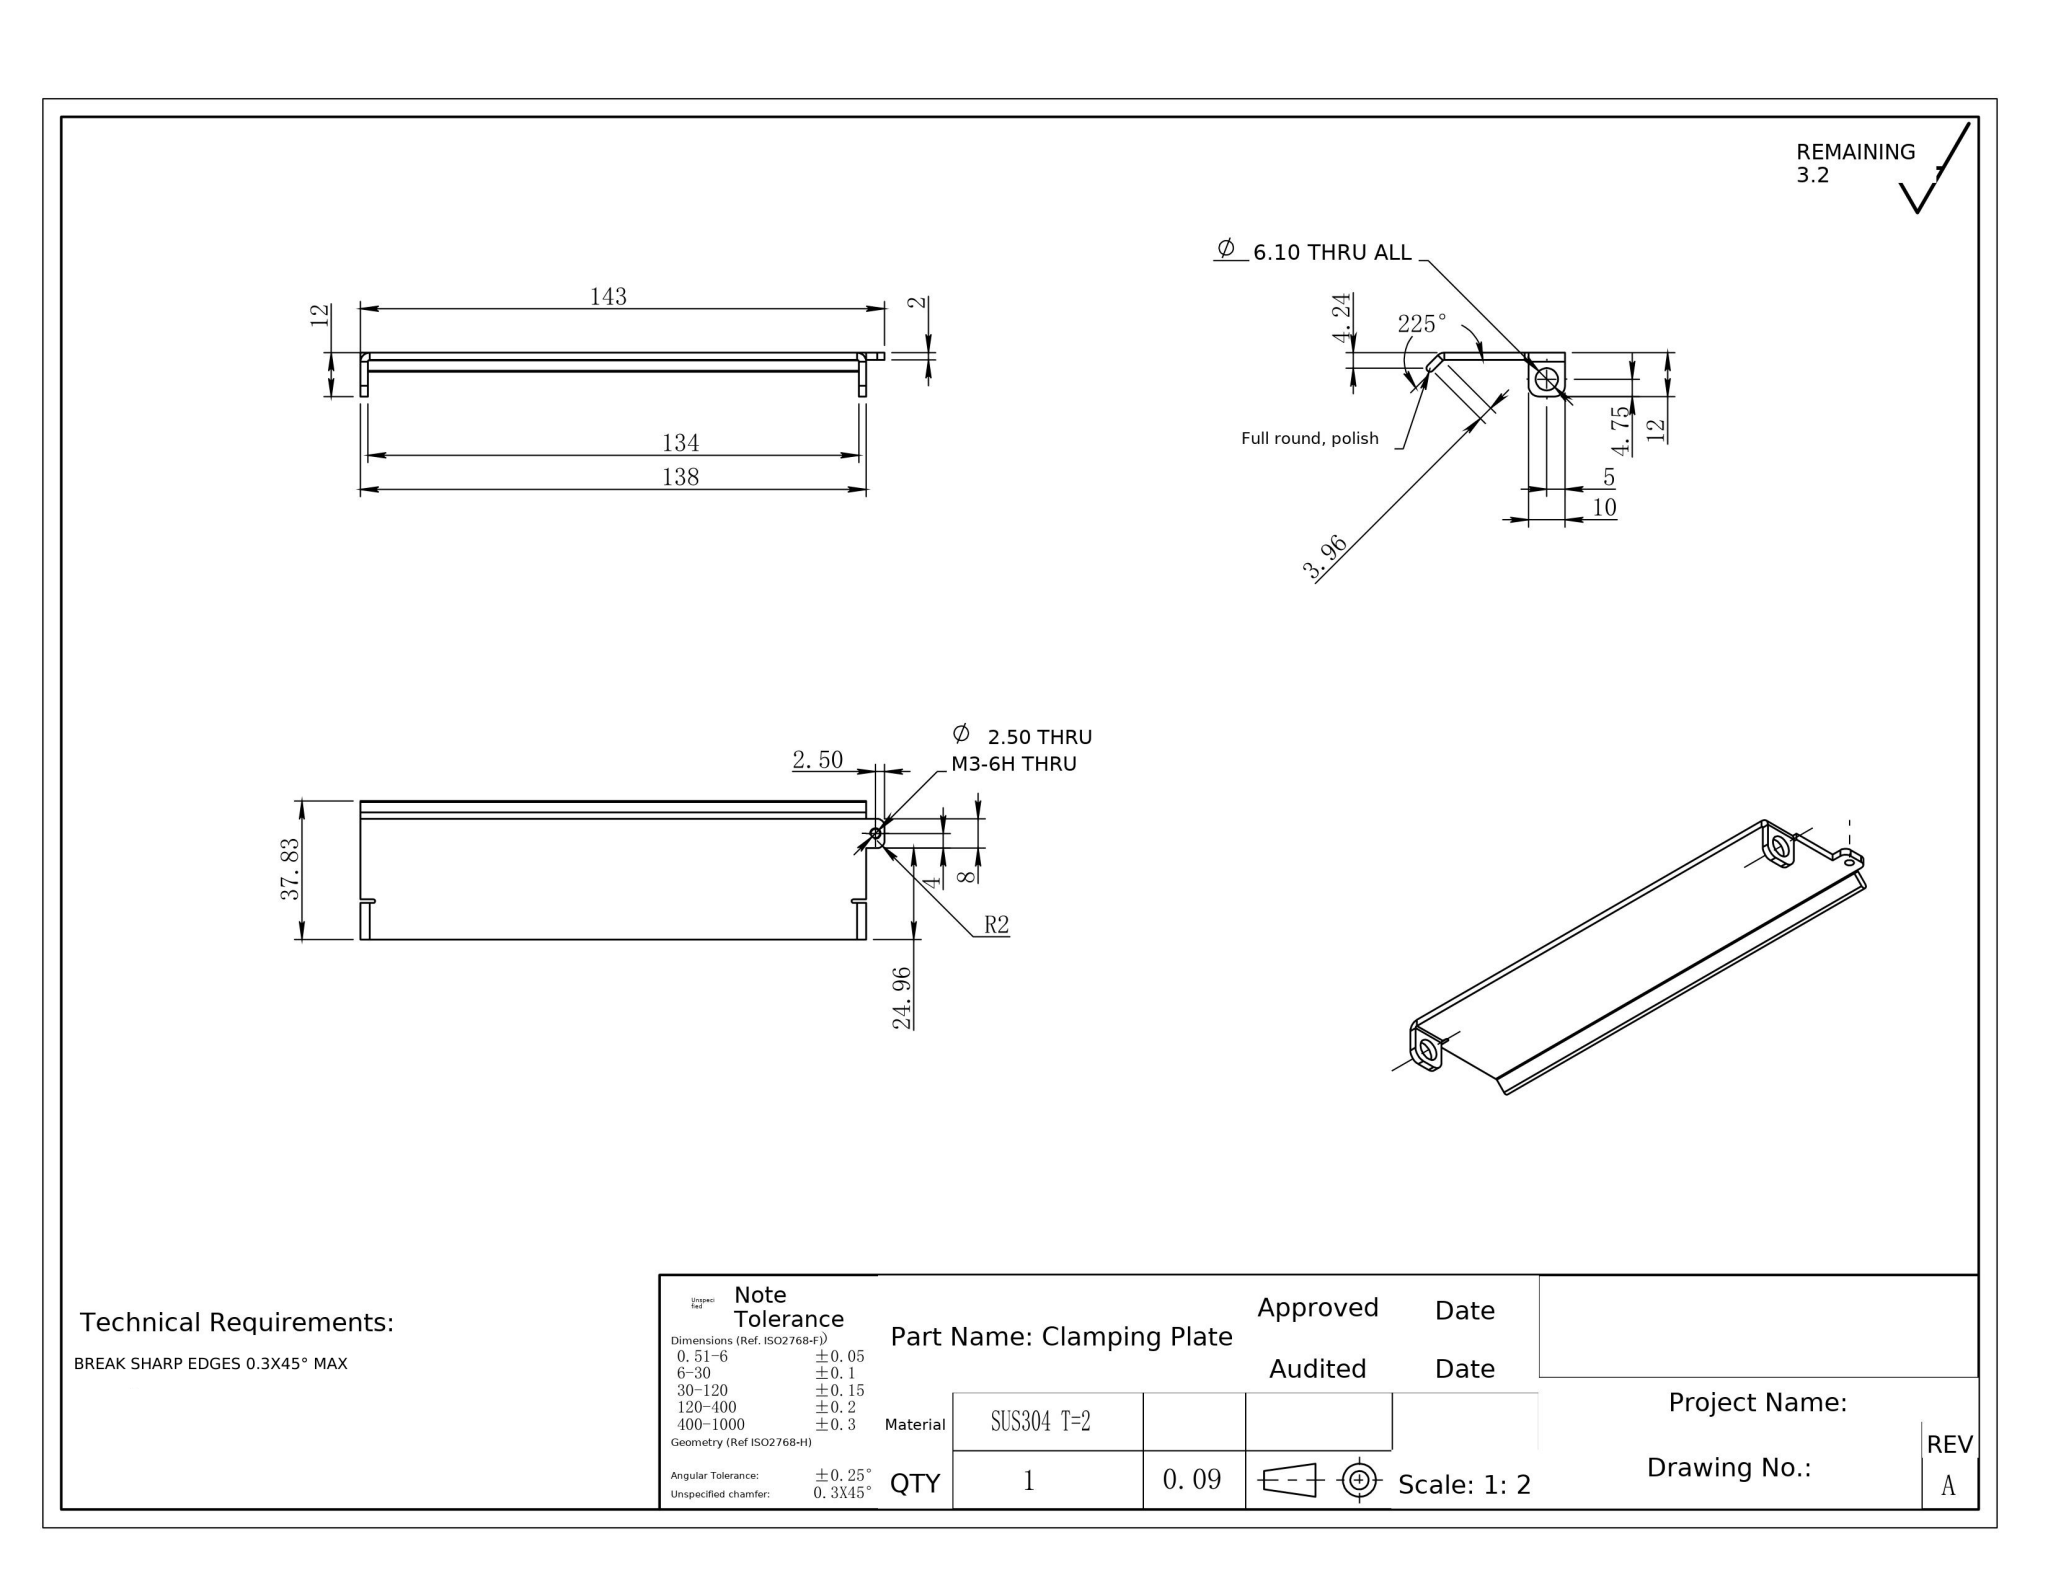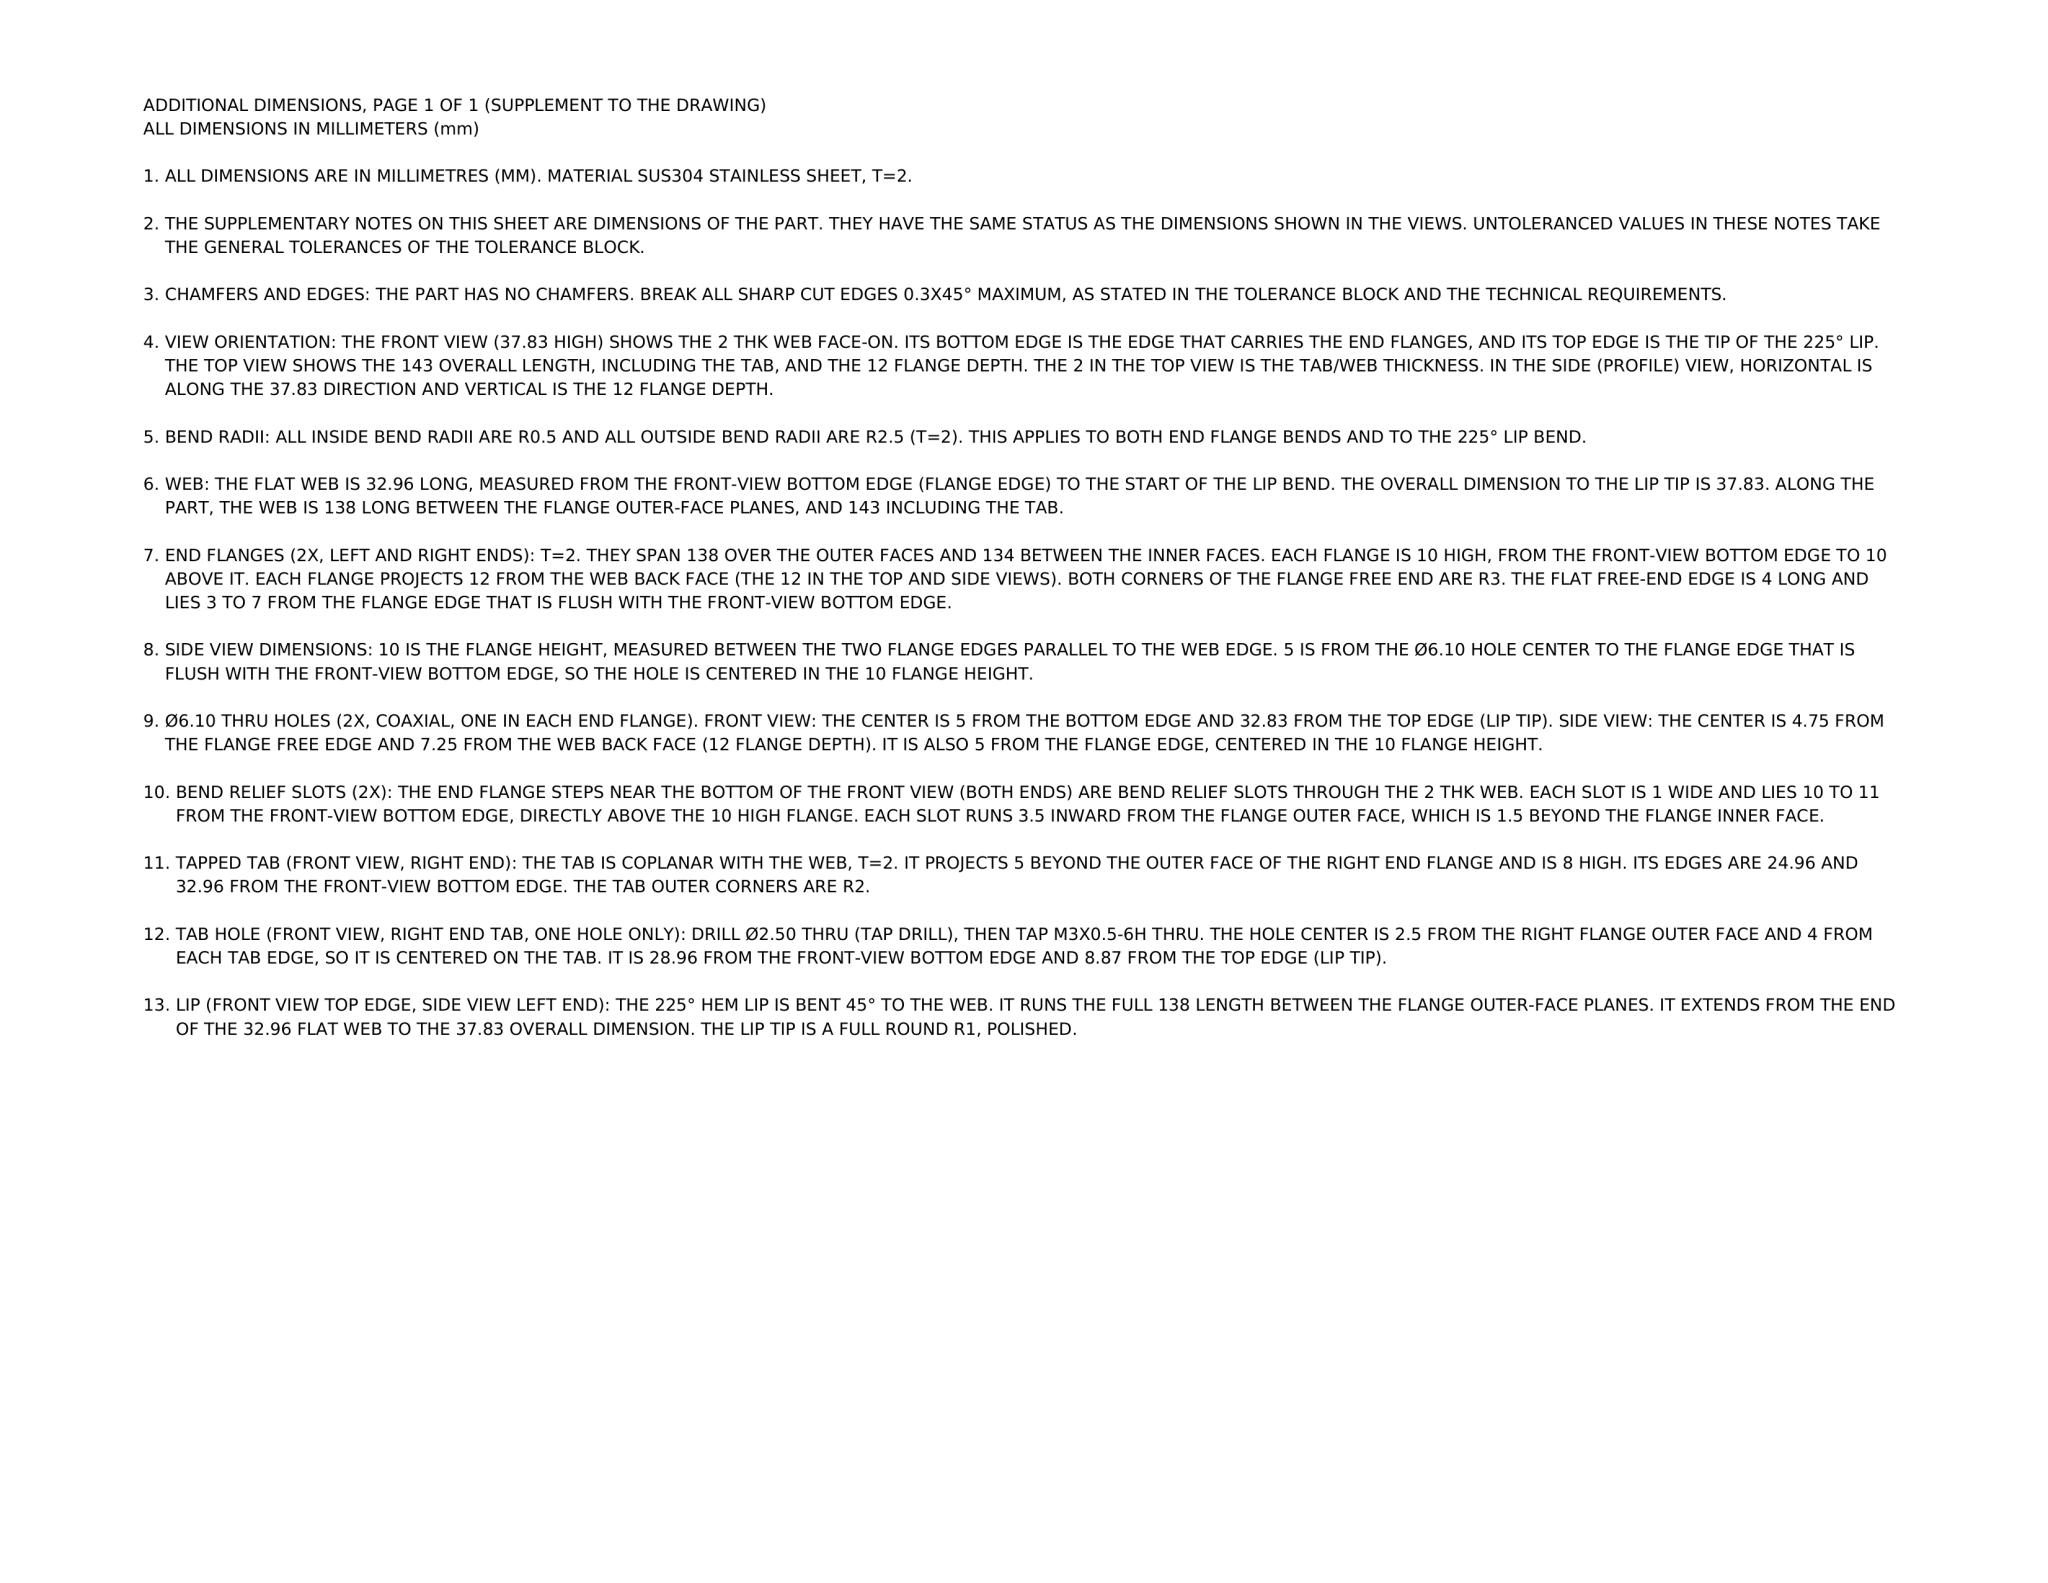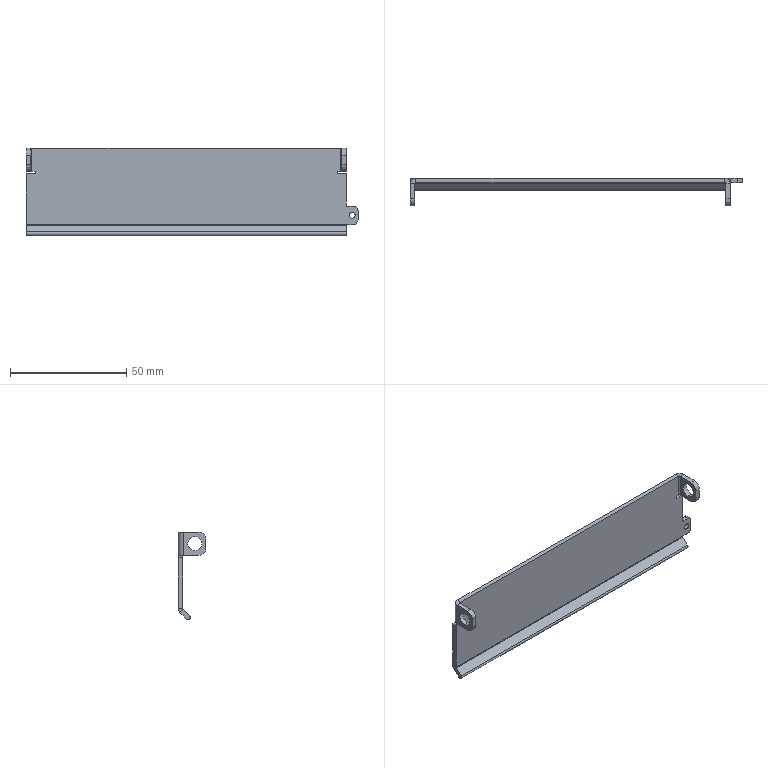Part | NX | mm | 1 solid | 54 faces | box 143 x 12 x 37.83 mm | volume 11027 mm3 | plane 32 | cylinder 22 | commonest cylinder face diameters 1 x5 6.1 x4 6 x4 5 x3 2.5 x2 2 x2 4 x2